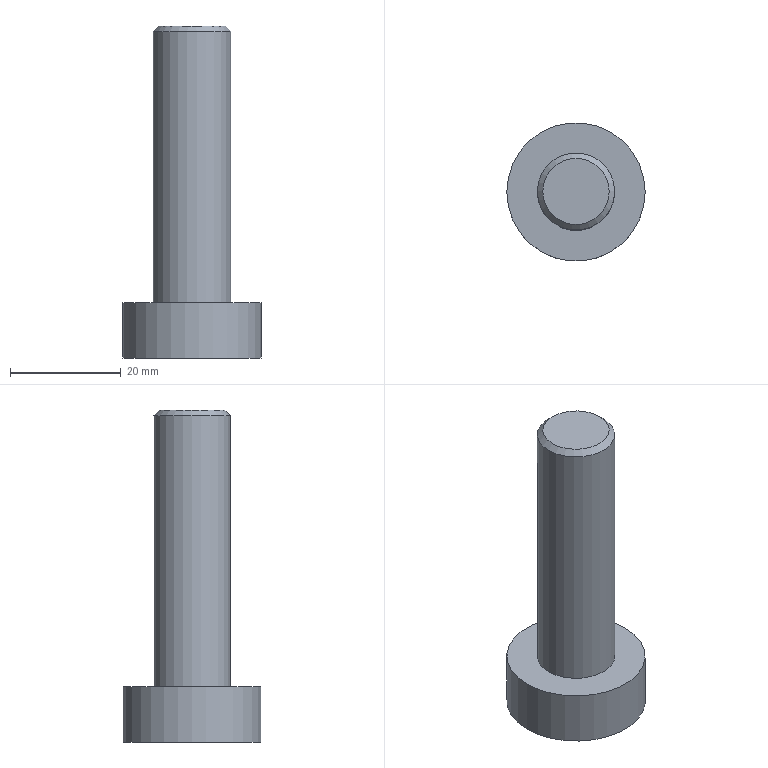Component | NX | TEMPLATE_LOCATING_SCREW | 1 solid | 19 faces | volume 10833 mm3 | plane 10 | cylinder 8 | cone 1 | commonest cylinder face diameters 2 x6 13.998 x1 25 x1